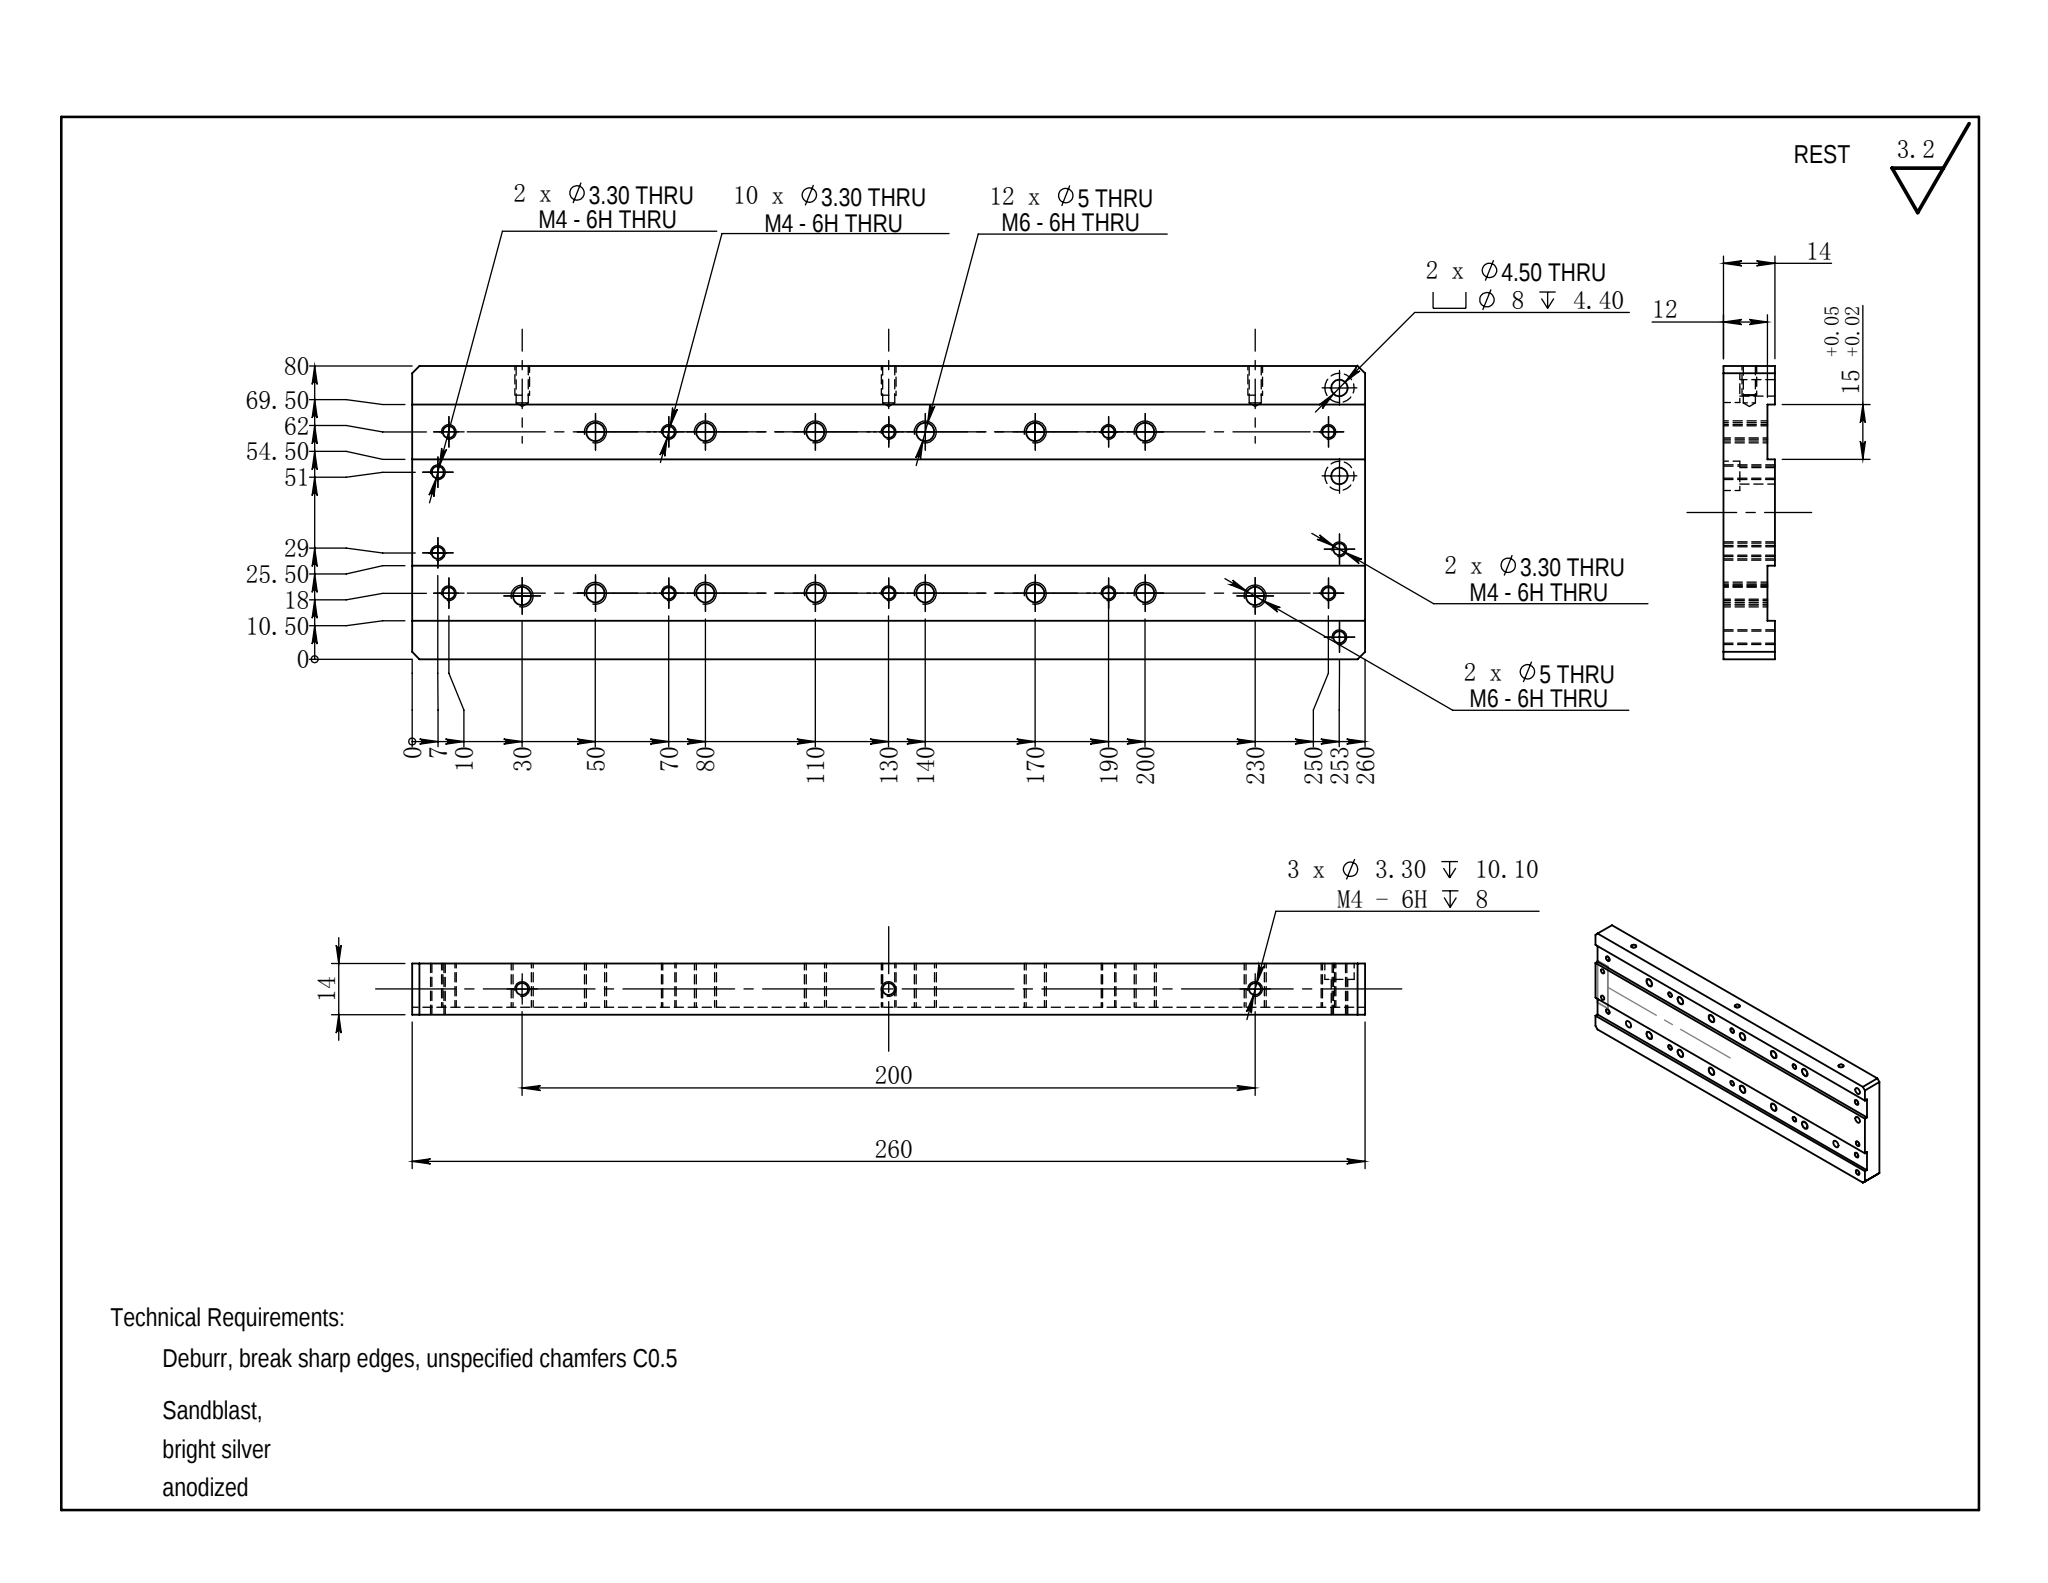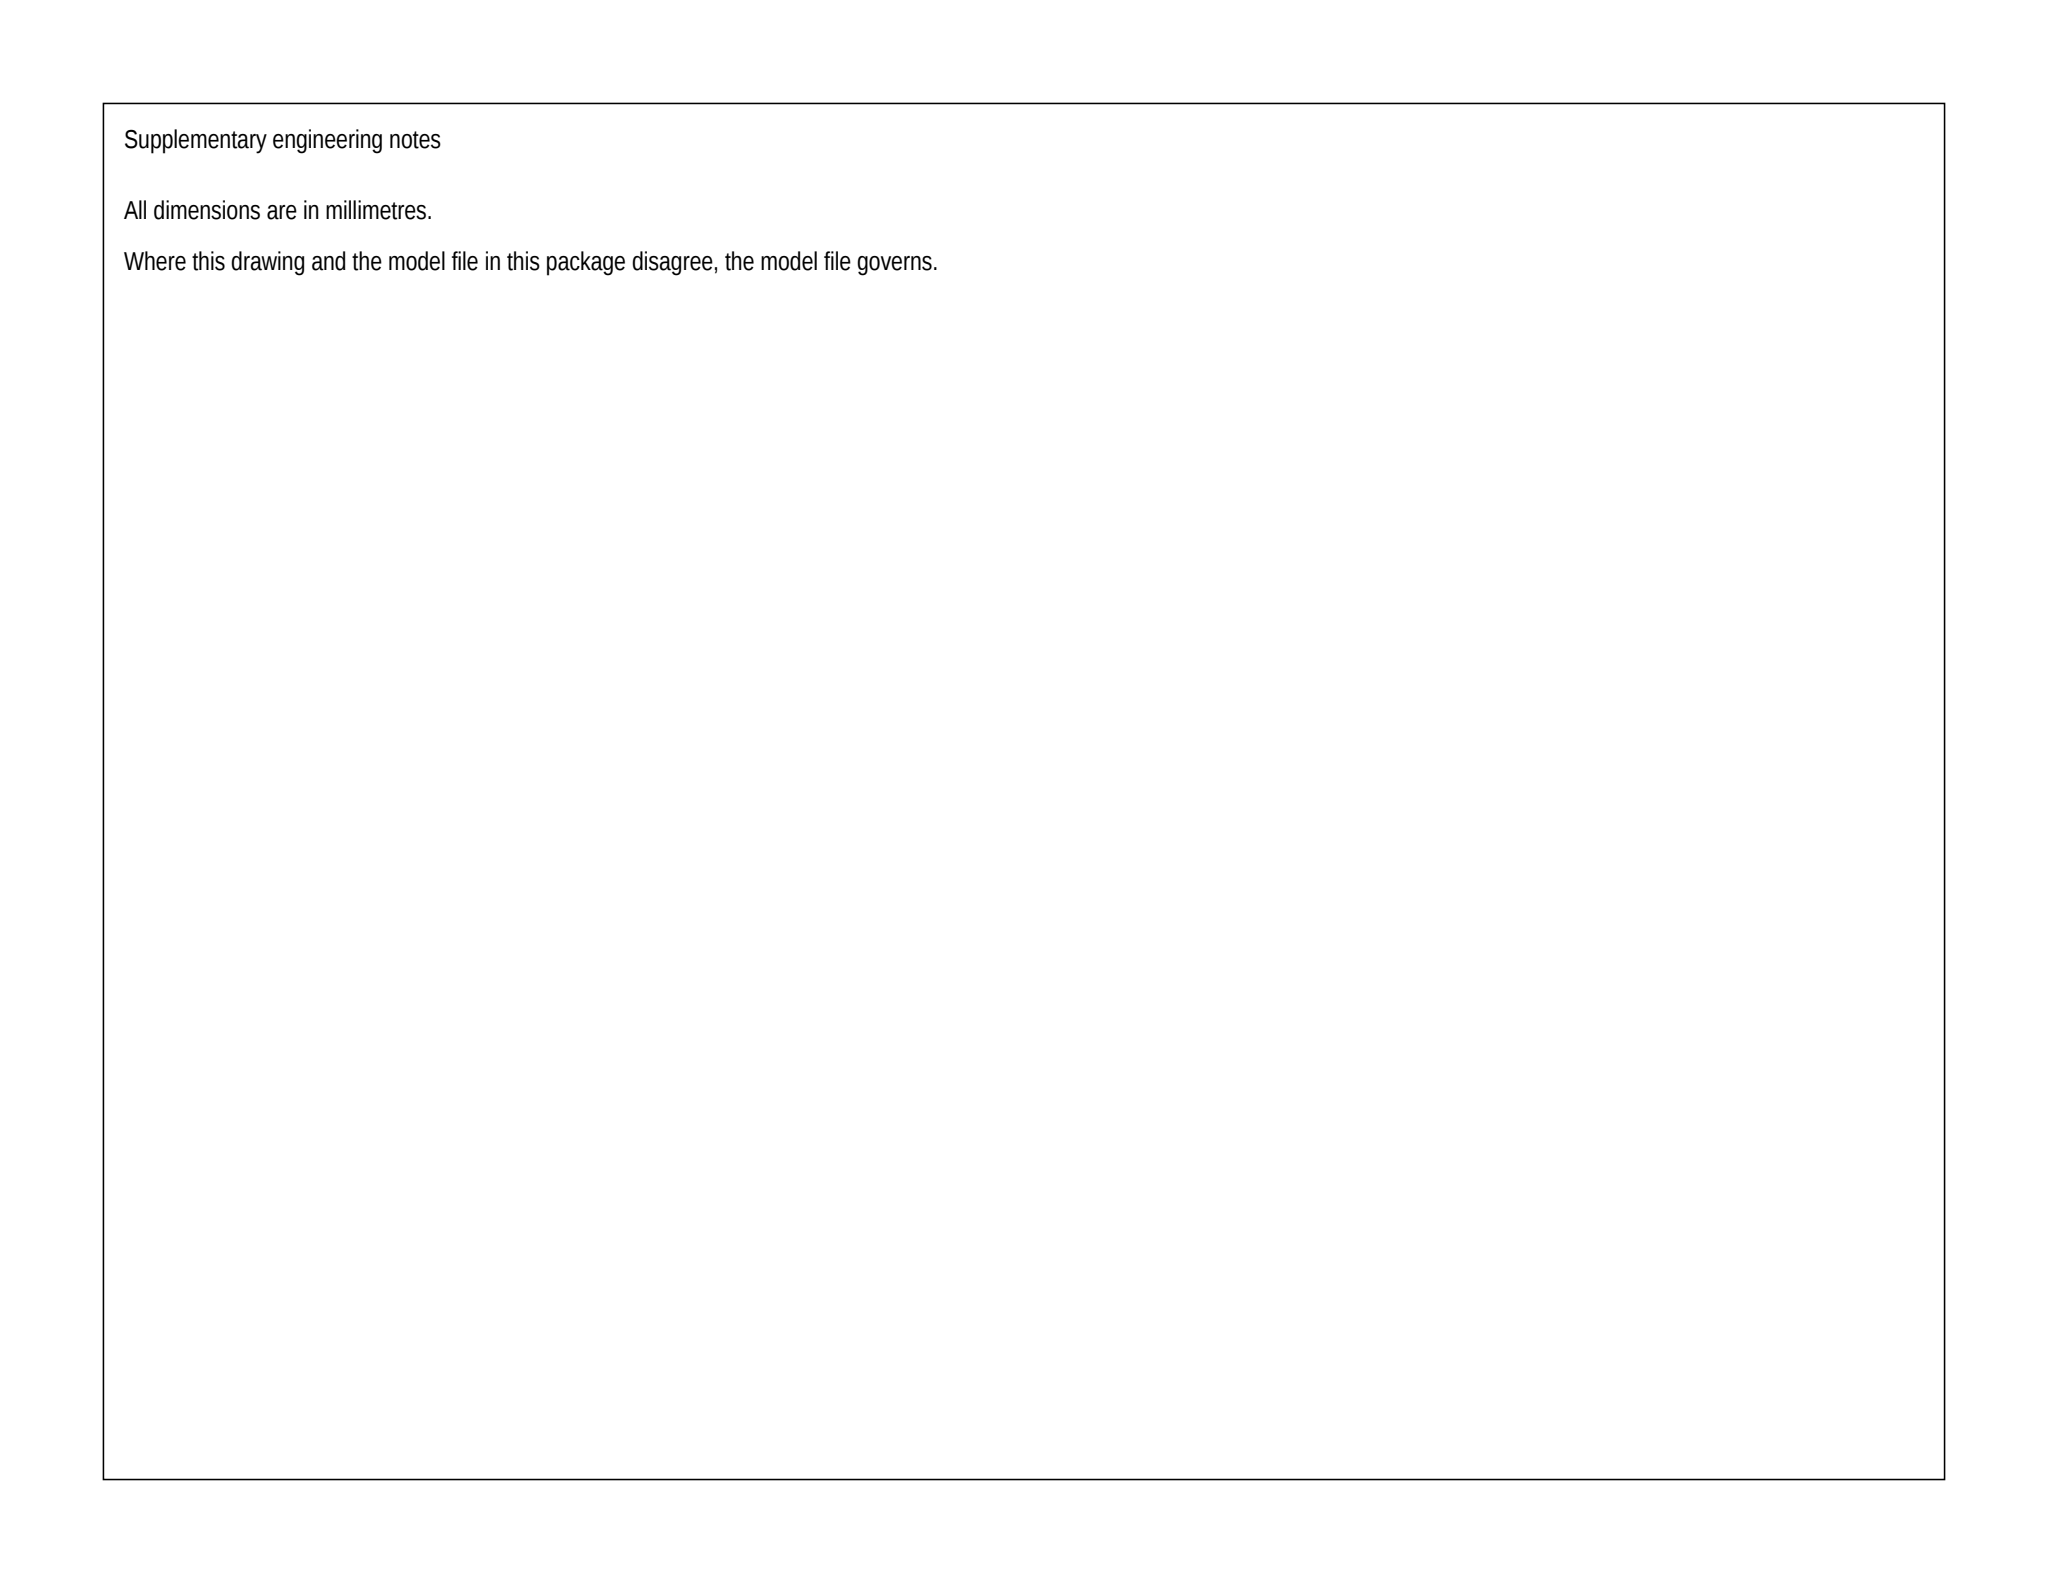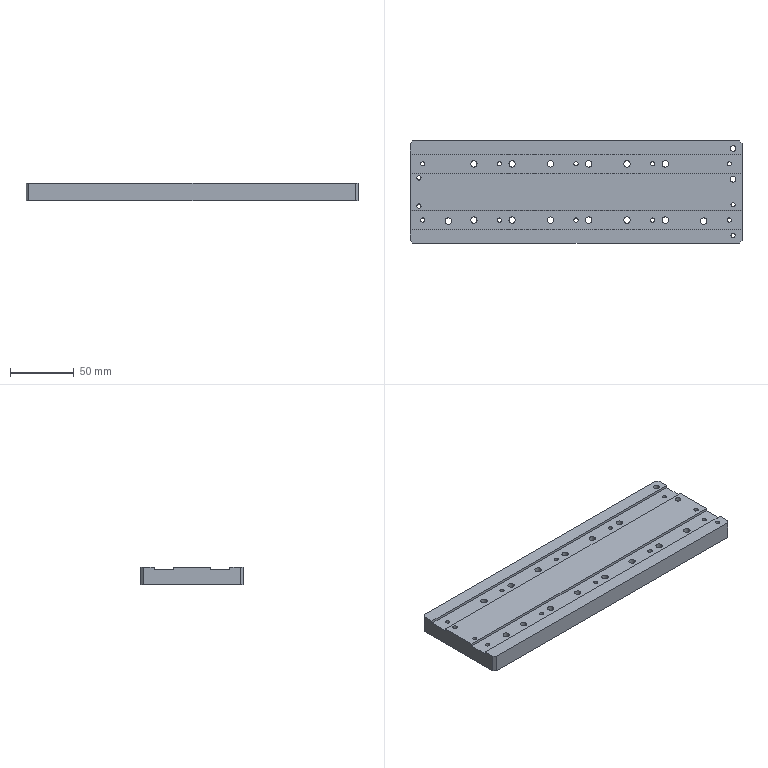Part | SolidWorks | mm | 1 solid | 96 faces | box 260 x 80 x 14 mm | volume 269669 mm3 | cylinder 70 | plane 20 | cone 6 | commonest cylinder face diameters 3.3 x34 5 x28 8 x4 4.5 x4
Drawing notes:
12X Ø5 FLAT-BOTTOM HOLE DP 12 (to recess floor, not thru 14 plate); rows Y=18 and Y=62, at X=50, 80, 110, 140, 170, 200 from bottom-left corner | from the solid: cylinders dia 5.0, axis z, positions (50/80/110/140/170/200, 18.0) and (…, 62.0), length 12.0
2X Ø5 HOLE DP 12 AT Y=17.25, X=30 AND X=230 from bottom-left corner (lower row offset from the Y=18 row) | from the solid: cylinders dia 5.0, axis z, pos (30.0, 17.25) and (230.0, 17.25), length 12.0
10X Ø3.3 HOLE DP 12 (not thru 14 plate); rows Y=18 and Y=62, at X=10, 70, 130, 190, 250 from bottom-left corner | from the solid: cylinders dia 3.3, axis z, positions (10/70/130/190/250, 18.0) and (…, 62.0), length 12.0
2X Ø3.3 THRU (14) AT X=7, Y=29 AND Y=51 from bottom-left corner | from the solid: cylinders dia 3.3, axis z, pos (7.0, 29.0) and (7.0, 51.0), length 14.0 = plate thickness
2X Ø3.3 THRU (14) AT X=253, Y=6 AND Y=30 from bottom-left corner | from the solid: cylinders dia 3.3, axis z, pos (253.0, 6.0) and (253.0, 30.0), length 14.0 = plate thickness
2X Ø4.5 THRU, C'BORE Ø8 DP 4.4 FROM TOP FACE, AT X=253, Y=50 AND Y=74 from bottom-left corner | from the solid: cylinders dia 4.5 length 9.6 and dia 8.0 length 4.4, axis z, pos (253.0, 50.0) and (253.0, 74.0); z-plane offset 4.4
PLATE 260 x 80 x 14; all hole X/Y locations measured from the bottom-left corner of the plate | from the solid: bbox_xyz [260.0, 80.0, 14.0], origin_note: positions from min corner of bbox
2X Ø3.30 THRU (14 thk) AT X=7 FROM LEFT END, Y=29 AND Y=51 FROM BOTTOM EDGE | from the solid: cylinders 3.3 axis z at [7,29] and [7,51], length 14.0 (= plate thickness 14)
10X Ø3.30 ▽12 (TO RECESS FLOOR) AT X=10, 70, 130, 190, 250 FROM LEFT END; Y=18 AND Y=62 FROM BOTTOM EDGE | from the solid: cylinders 3.3 axis z at [10/70/130/190/250, 18] and [...,62], length 12.0; z-plane at 12.0
12X Ø5 ▽12 (TO RECESS FLOOR) AT X=50, 80, 110, 140, 170, 200 FROM LEFT END; Y=18 AND Y=62 FROM BOTTOM EDGE | from the solid: cylinders 5.0 axis z at [50/80/110/140/170/200, 18] and [...,62], length 12.0
2X Ø5 ▽12 AT X=30 AND X=230 FROM LEFT END, Y=17.25 FROM BOTTOM EDGE | from the solid: cylinders 5.0 axis z at [30,17.25] and [230,17.25], length 12.0
2X Ø3.30 THRU (14 thk) AT X=253 FROM LEFT END, Y=6 AND Y=30 FROM BOTTOM EDGE | from the solid: cylinders 3.3 axis z at [253,6] and [253,30], length 14.0
2X Ø4.50 THRU, C'BORE Ø8 ▽4.40 FROM TOP FACE, AT X=253 FROM LEFT END, Y=50 AND Y=74 FROM BOTTOM EDGE | from the solid: cylinders 4.5 axis z at [253,50] and [253,74] length 9.6 with coaxial 8.0 length 4.4; z-plane at 4.4 (4.4+9.6=14 thk)
3X Ø3.30 ▽10.10 IN SIDE FACE AT X=30, 130, 230 FROM LEFT END, Z=7 FROM BOTTOM FACE | from the solid: cylinders 3.3 axis y at [30,null,7], [130,null,7], [230,null,7], length 10.1
14X M6-6H THREAD IN Ø5 TAP-DRILL HOLES ▽12 (TO RECESS FLOOR, NOT THRU 14 PLATE): 12X AT Y=18 AND Y=62, X=50, 80, 110, 140, 170, 200; 2X AT Y=17.25, X=30 AND 230 - ALL FROM BOTTOM-LEFT CORNER OF PLATE | from the solid: cylinders dia 5.0 axis z length 12.0 at (50/80/110/140/170/200, 18 and 62) and (30, 17.25), (230, 17.25); plate bbox 260x80x14 with z plane at 12.0
14X M6-6H THREAD IN Ø5 TAP-DRILL HOLES ▽12 (TO RECESS FLOOR, NOT THRU 14 PLATE): 12X AT Y=18 AND Y=62, X=50, 80, 110, 140, 170, 200; 2X AT Y=17.25, X=30 AND 230 — ALL FROM BOTTOM-LEFT CORNER OF PLATE | from the solid: cylinders dia 5.0 axis z, length 12.0 at (50/80/110/140/170/200, 18 and 62) and (30, 17.25) and (230, 17.25); bbox 260x80x14
14X M6-6H TAPPED HOLE: Ø5 TAP DRILL ▽12 FROM RECESS FACE (NOT THRU 14 PLATE) - 12X AT Y=18 AND Y=62, X=50, 80, 110, 140, 170, 200; 2X AT Y=17.3, X=30 AND X=230, ALL FROM BOTTOM-LEFT CORNER | from the solid: cylinders: 14X hole/bore dia 5.0 axis z from 0.0 to 12.0 at (50/80/110/140/170/200, 18 & 62) and (30/230, 17.3)
4X CHAMFER 2 x 45° (C2) ON VERTICAL CORNER EDGES AT X=0 & X=260 / Y=0 & Y=80, FULL 14 THICKNESS | from the solid: inclined_planes: four 45°/45° faces, size [2.0,2.0,14.0] at bbox_from [0,0,0], [0,78,0], [258,0,0], [258,78,0]
14X M6-6H TAPPED HOLE, Ø5 TAP DRILL ▽12 FROM RECESS FLOOR (NOT THRU 14 PLATE): 12X AT Y=18 AND Y=62, X=50, 80, 110, 140, 170, 200; 2X AT Y=17.3, X=30 AND X=230 - ALL FROM BOTTOM-LEFT CORNER (replaces garbled M6 callout) | from the solid: cylinders: Ø5.0 z-axis holes from 0.0 to 12.0 at (50,18),(50,62),(80,18),(80,62),(110,18),(110,62),(140,18),(140,62),(170,18),(170,62),(200,18),(200,62),(30,17.3),(230,17.3)
build123d program:
from build123d import *

# Parameters (mm, degrees)
SKETCH1_W                                       = 260
SKETCH1_H                                       = 80
BOSS_EXTRUDE1_DEPTH                             = 7
CHAMFER1_SIZE                                   = 2
SKETCH2_W                                       = 260
SKETCH2_H                                       = 15
CUT_EXTRUDE1_DEPTH                              = 2
M4_TAPPED_HOLE6_D                               = 3.3
M4_TAPPED_HOLE1_D                               = 3.3
M4_TAPPED_HOLE1_DEPTH                           = 10.1
M4_TAPPED_HOLE1_TIP                             = 0.9914
LPATTERN1_COUNT                                 = 5
LPATTERN1_PITCH                                 = 60
M4_TAPPED_HOLE5_D                               = 3.3
M4_TAPPED_HOLE7_D                               = 3.3
M6_TAPPED_HOLE1_D                               = 5
LPATTERN2_COUNT                                 = 6
LPATTERN2_PITCH                                 = 30
M6_TAPPED_HOLE2_D                               = 5
M4_HEX_SOCKET_HEAD_CAP_SCREW_CBORE1_D           = 4.5
M4_HEX_SOCKET_HEAD_CAP_SCREW_CBORE1_CBORE_D     = 8
M4_HEX_SOCKET_HEAD_CAP_SCREW_CBORE1_CBORE_DEPTH = 4.4


with BuildPart() as part:
    # Sketch1 → Boss-Extrude1 (new, symmetric)
    with BuildSketch(Plane.XY):
        Rectangle(SKETCH1_W, SKETCH1_H)
    extrude(amount=BOSS_EXTRUDE1_DEPTH, both=True)

    # Chamfer1
    chamfer1_edges = [part.edges().sort_by_distance(p)[0] for p in [
        (130, -40, 0),
        (-130, -40, 0),
        (-130, 40, 0),
        (130, 40, 0),
    ]]
    chamfer(chamfer1_edges, length=CHAMFER1_SIZE)

    # Sketch2 → Cut-Extrude1 (cut)
    with BuildSketch(Plane.XY.offset(7)):
        with Locations((0, 22)):
            Rectangle(SKETCH2_W, SKETCH2_H)
        with Locations((0, -22)):
            Rectangle(SKETCH2_W, SKETCH2_H)
    extrude(amount=-CUT_EXTRUDE1_DEPTH, mode=Mode.SUBTRACT)

    # M4 Tapped Hole6 (through all)
    with Locations(Plane.XY.offset(5)):
        with Locations((120, 22), (120, -22)):
            m4_tapped_hole6 = Hole(M4_TAPPED_HOLE6_D / 2)

    # M4 Tapped Hole1
    with Locations(Plane(origin=(78.356, 40, 6.896), x_dir=(-1, 0, 0), z_dir=(0, 1, 0))):
        with Locations((-21.644, -6.896), (78.356, -6.896), (178.356, -6.896)):
            Hole(M4_TAPPED_HOLE1_D / 2, depth=M4_TAPPED_HOLE1_DEPTH)
            with Locations((0, 0, -(M4_TAPPED_HOLE1_DEPTH + M4_TAPPED_HOLE1_TIP / 2))):  # 118° drill point
                Cone(0, M4_TAPPED_HOLE1_D / 2, M4_TAPPED_HOLE1_TIP, mode=Mode.SUBTRACT)

    # LPattern1: M4 Tapped Hole6 ×5
    with Locations(*[(-i * LPATTERN1_PITCH, 0, 0) for i in range(1, LPATTERN1_COUNT)]):
        add(m4_tapped_hole6, mode=Mode.SUBTRACT)

    # M4 Tapped Hole5 (through all)
    with Locations(Plane(origin=(0, 0, -7), x_dir=(-1, 0, 0), z_dir=(0, 0, -1))):
        with Locations((123, 11), (123, -11)):
            Hole(M4_TAPPED_HOLE5_D / 2)

    # M4 Tapped Hole7 (through all)
    with Locations(Plane.XY.offset(7)):
        with Locations((123, -10), (123, -34)):
            Hole(M4_TAPPED_HOLE7_D / 2)

    # M6 Tapped Hole1 (through all)
    with Locations(Plane.XY.offset(7)):
        with Locations((70, 22), (70, -22)):
            m6_tapped_hole1 = Hole(M6_TAPPED_HOLE1_D / 2)

    # LPattern2: M6 Tapped Hole1 ×6
    with Locations(*[(-i * LPATTERN2_PITCH, 0, 0) for i in range(1, LPATTERN2_COUNT)]):
        add(m6_tapped_hole1, mode=Mode.SUBTRACT)

    # M6 Tapped Hole2 (through all)
    with Locations(Plane(origin=(0, 0, -7), x_dir=(-1, 0, 0), z_dir=(0, 0, -1))):
        with Locations((-100, -22.75), (100, -22.75)):
            Hole(M6_TAPPED_HOLE2_D / 2)

    # M4 Hex Socket Head Cap Screw CBORE1 (through all)
    with Locations(Plane(origin=(0, 0, -7), x_dir=(-1, 0, 0), z_dir=(0, 0, -1))):
        with Locations((-123, 34), (-123, 10)):
            CounterBoreHole(M4_HEX_SOCKET_HEAD_CAP_SCREW_CBORE1_D / 2, M4_HEX_SOCKET_HEAD_CAP_SCREW_CBORE1_CBORE_D / 2, M4_HEX_SOCKET_HEAD_CAP_SCREW_CBORE1_CBORE_DEPTH)


solid = part.part